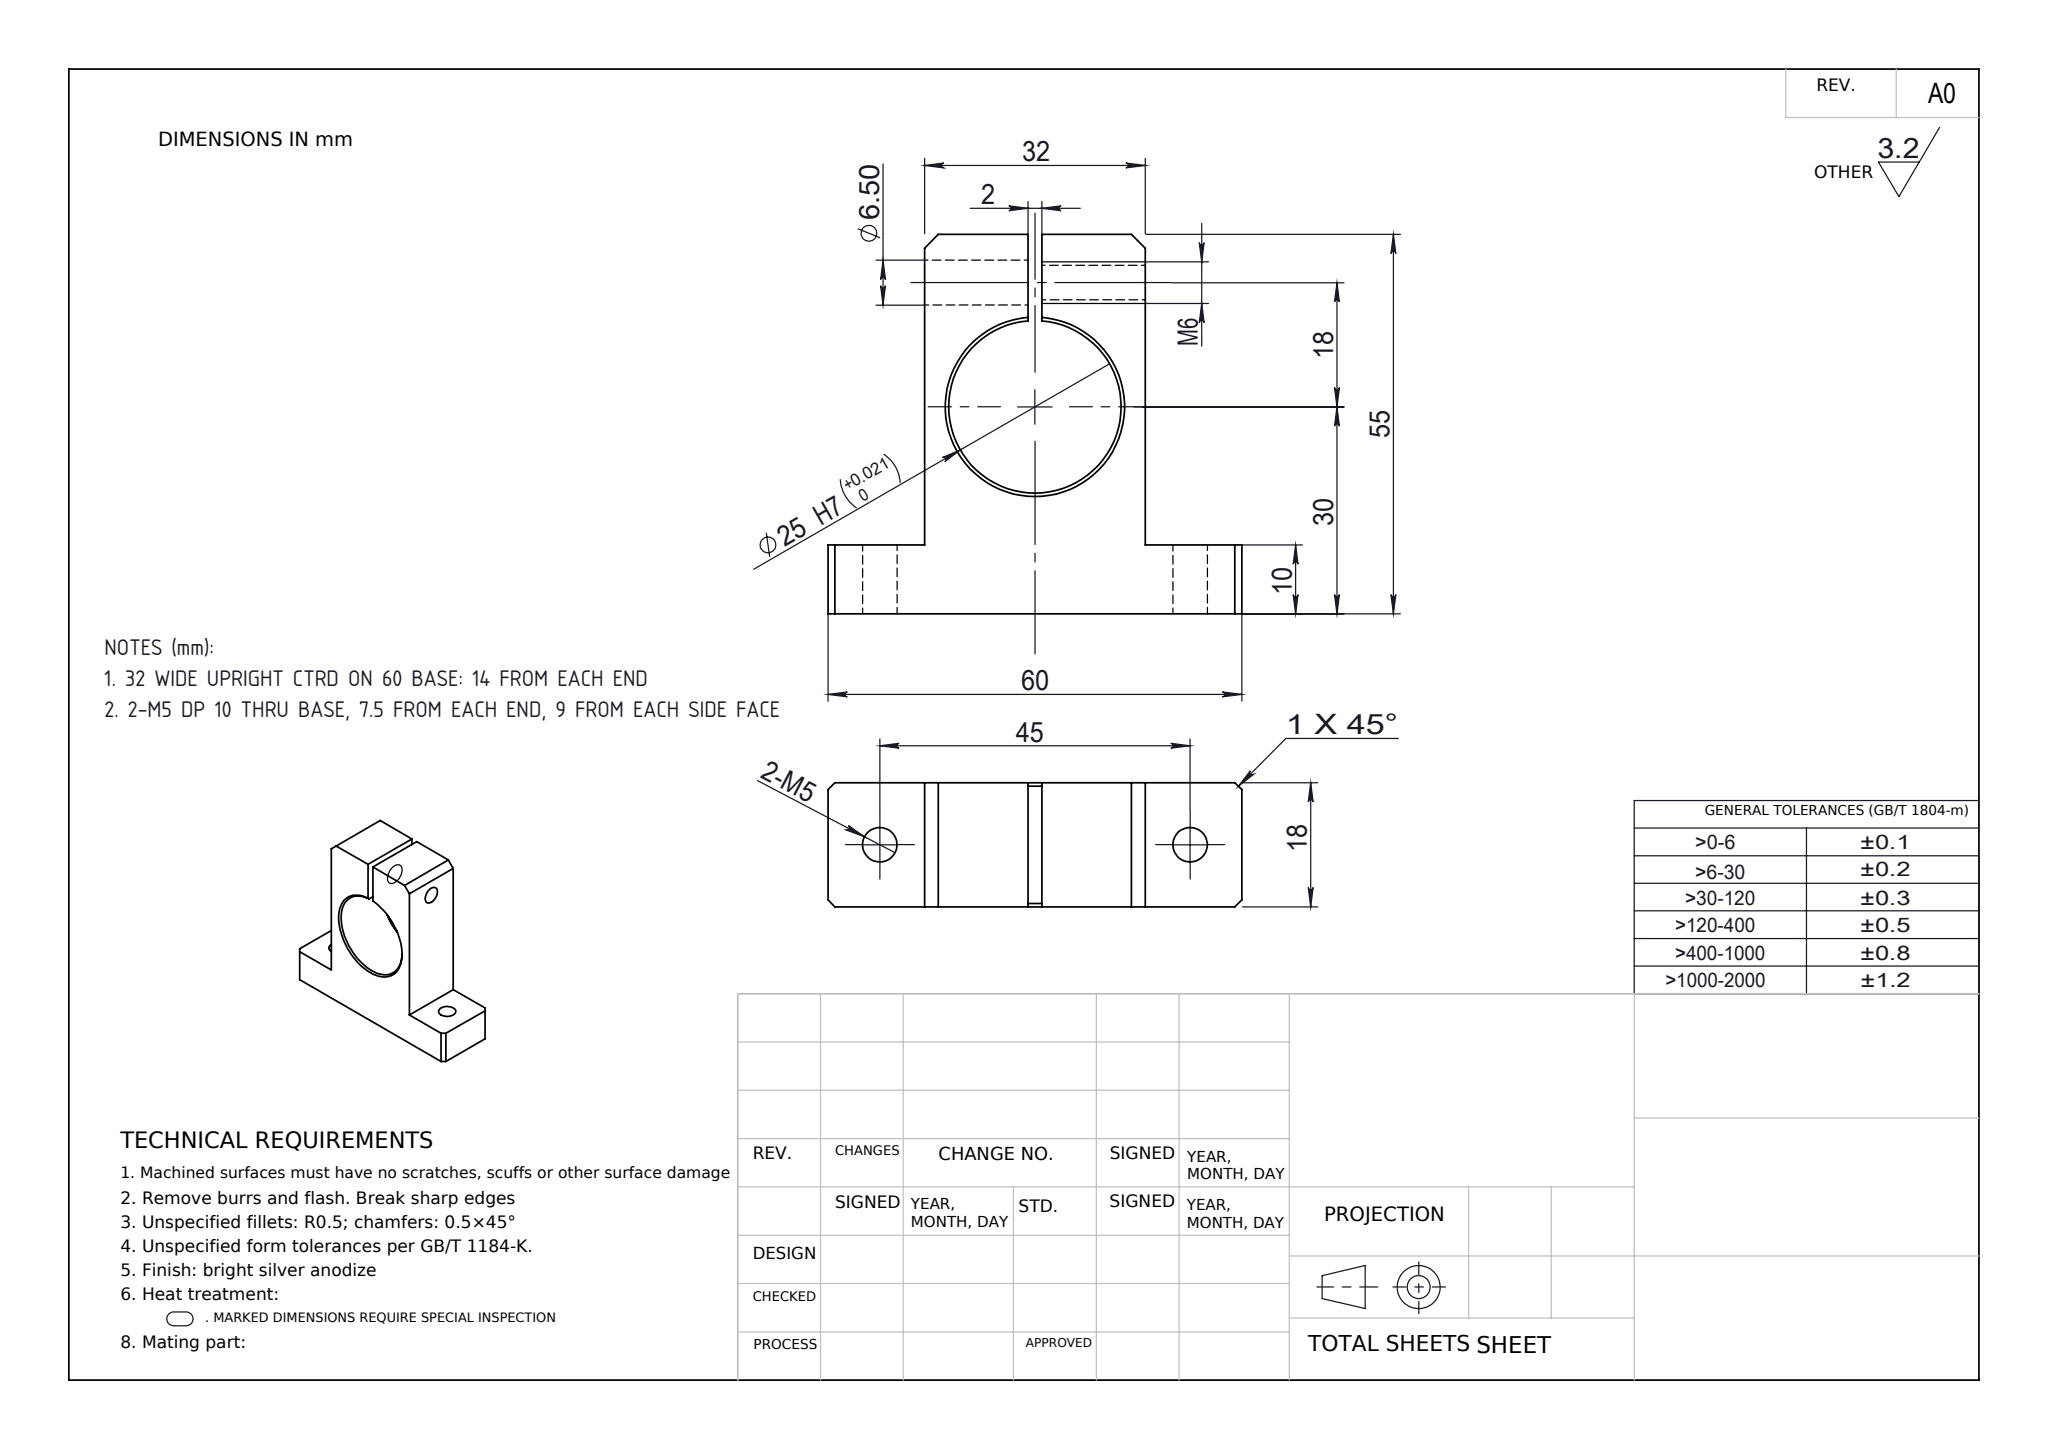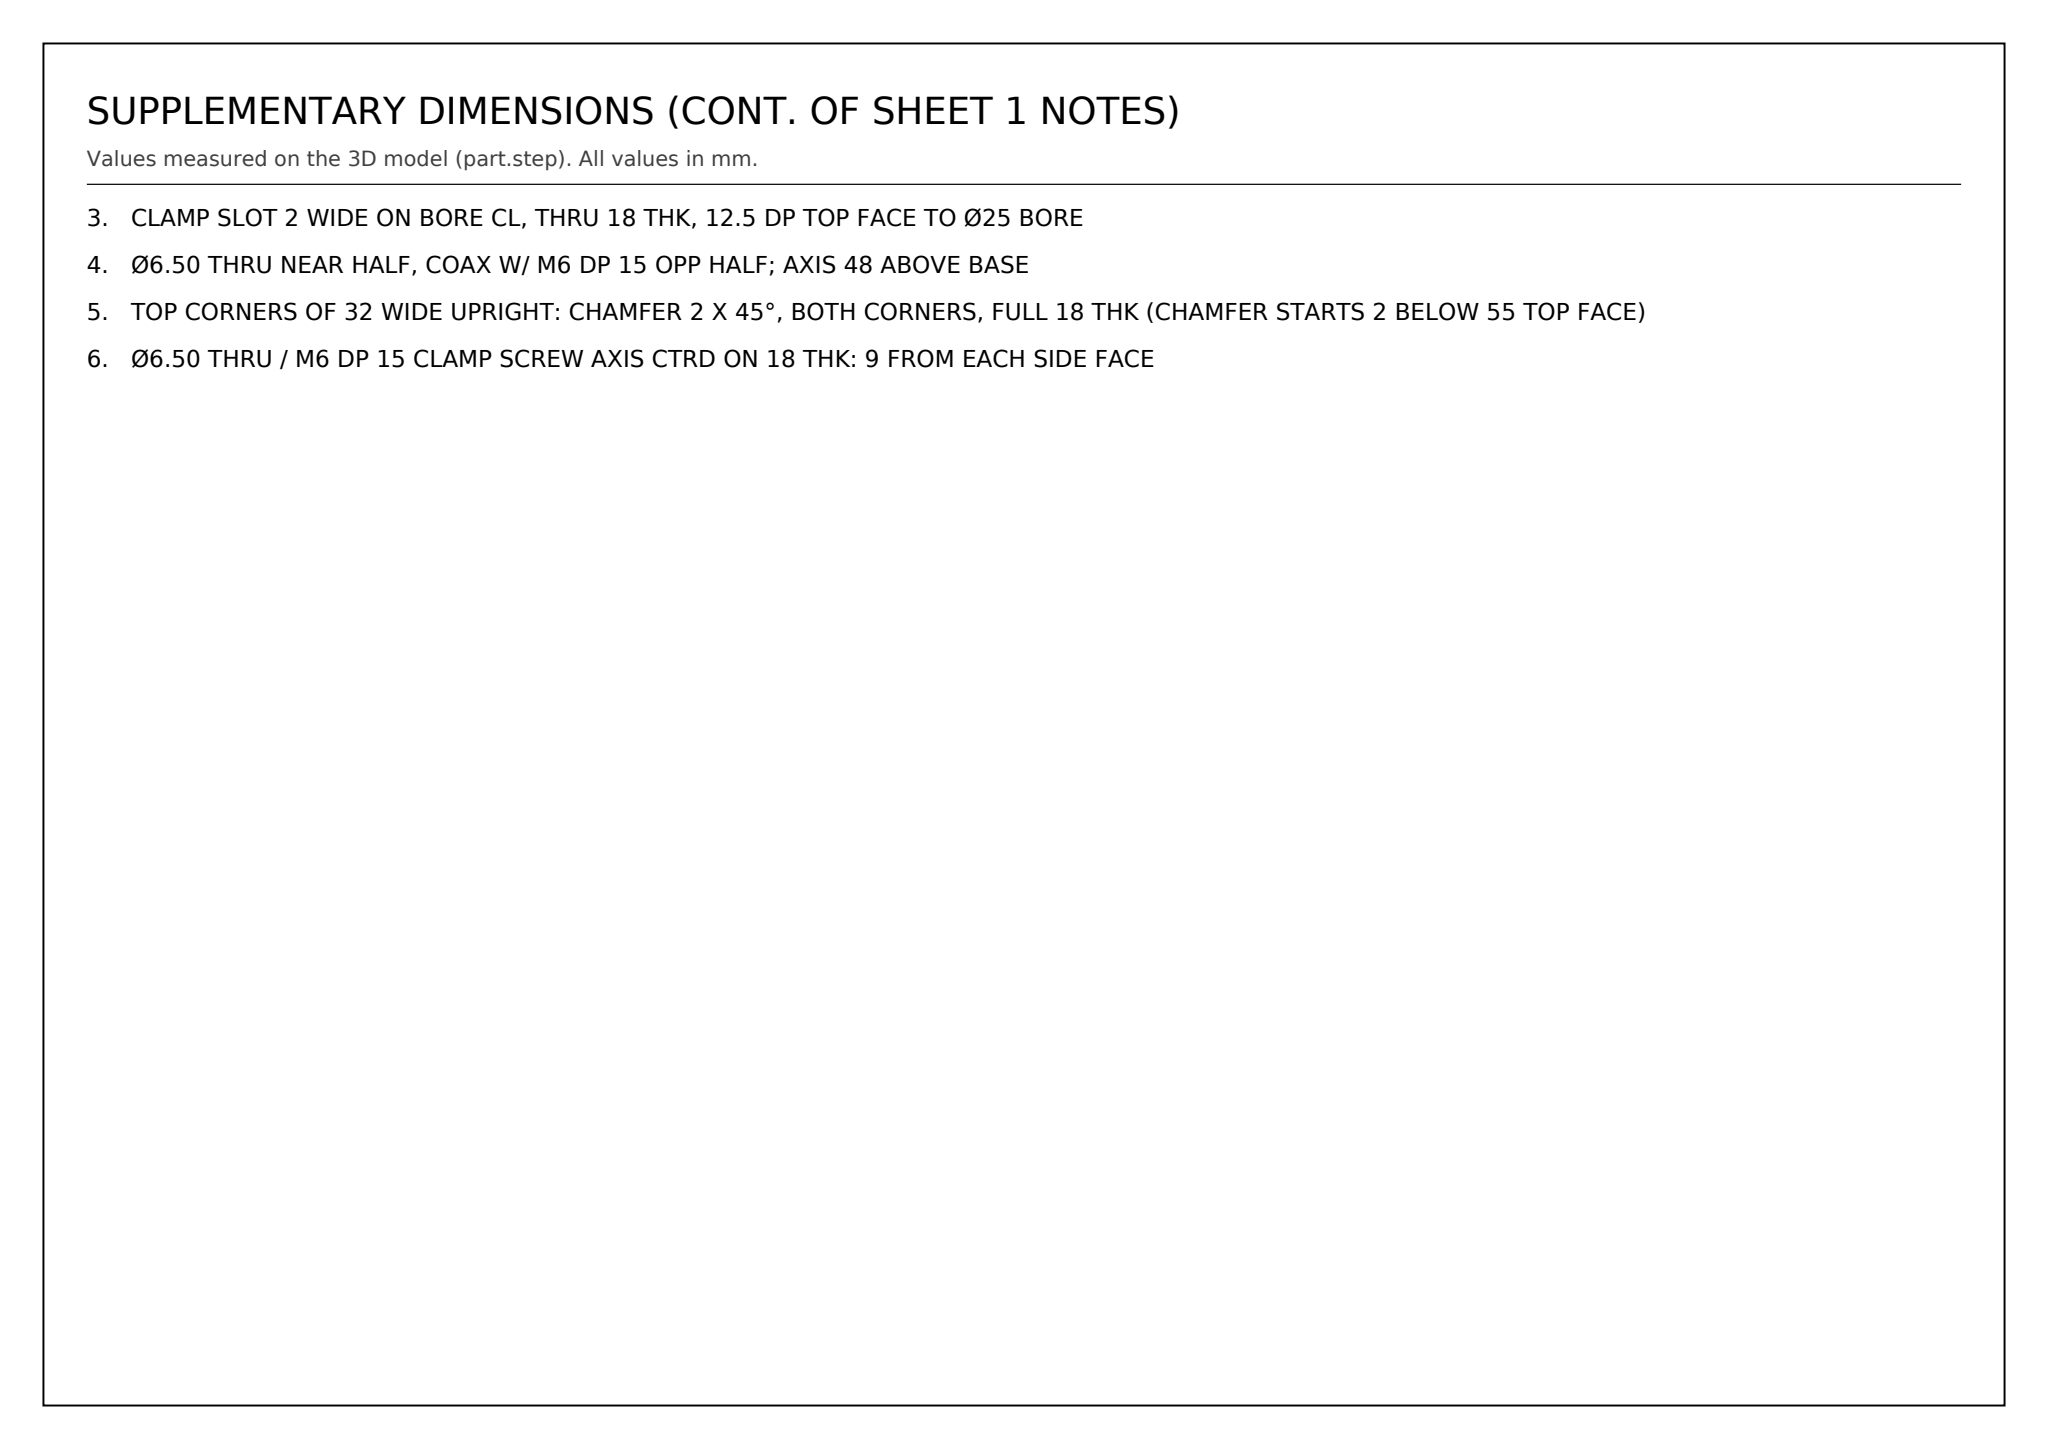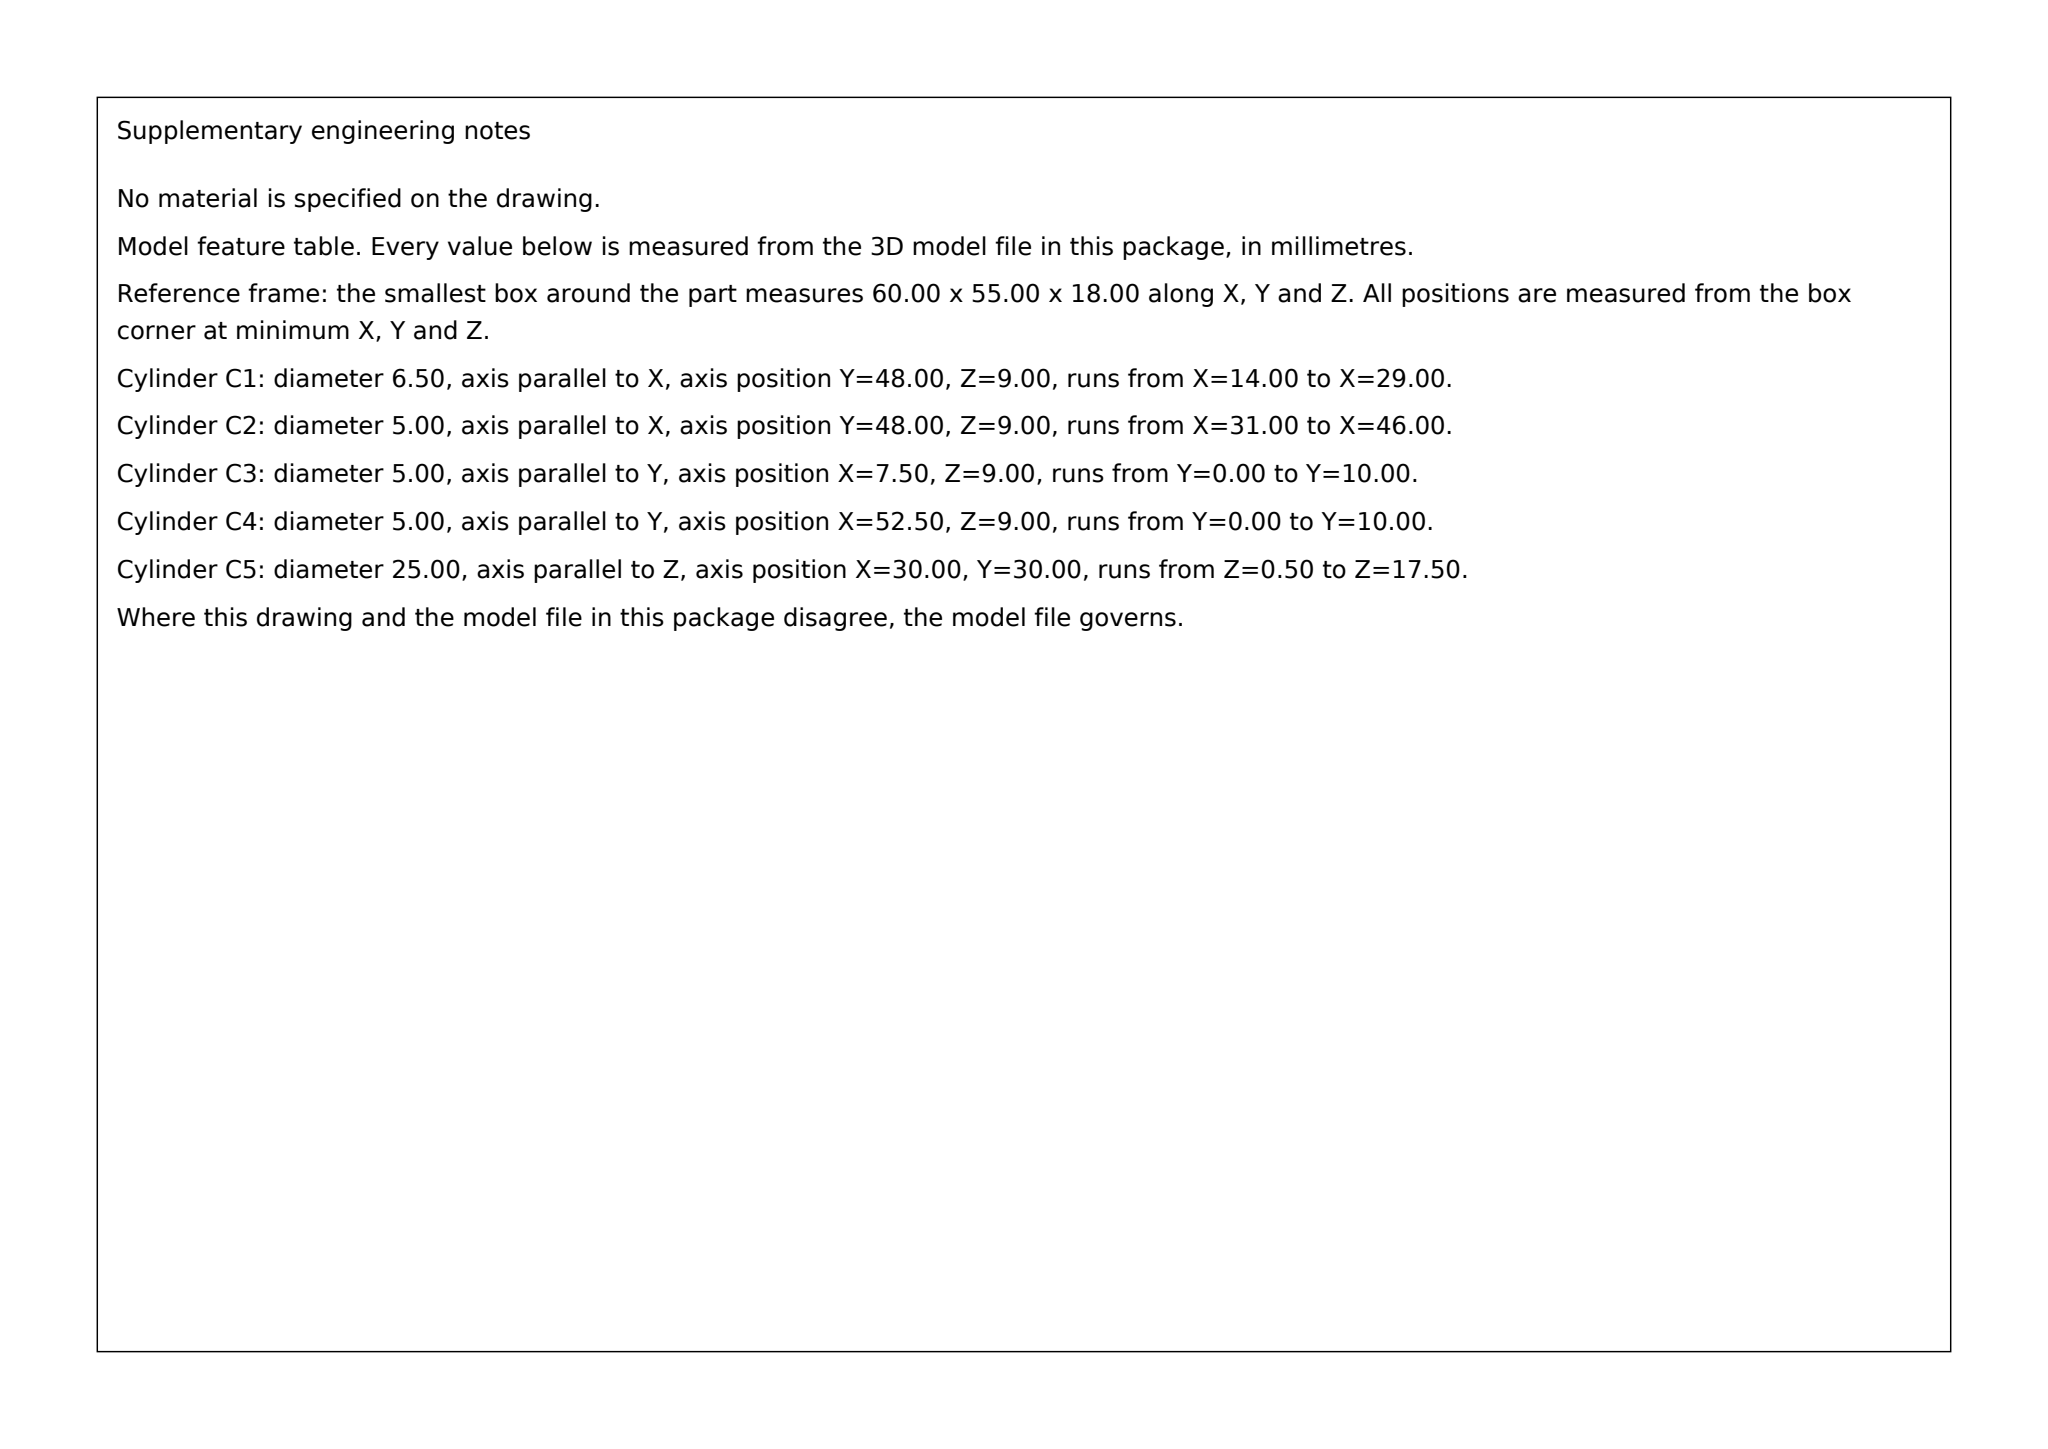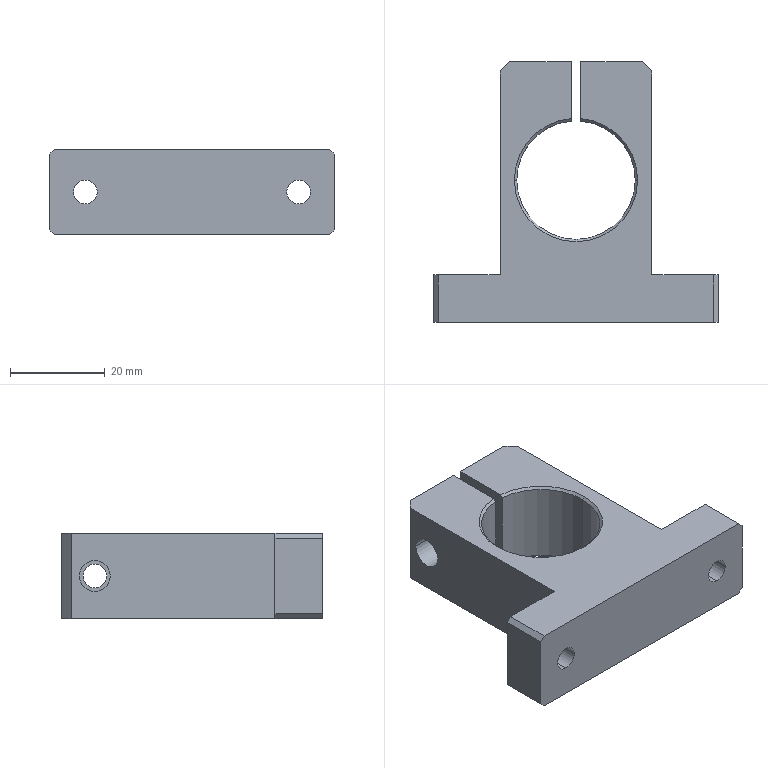Part | SolidWorks | mm | 1 solid | 36 faces | box 60 x 55 x 18 mm | volume 26137 mm3 | plane 19 | cylinder 11 | cone 6 | commonest cylinder face diameters 5 x6 25 x3 6.5 x2
Drawing notes:
32 WIDE UPRIGHT CTRD ON 60 BASE: 14 FROM EACH END | from the solid: x-planes at 14 and 46 vs bbox x 0-60
2-M5 DP 10 THRU BASE, 7.5 FROM EACH END, 9 FROM EACH SIDE FACE | from the solid: cyl Ø5 axis y at x=7.5 & x=52.5, z=9, length 10; base 60 long x 18 wide
CLAMP SLOT 2 WIDE ON BORE CL, THRU 18 THK, 12.5 DP TOP FACE TO Ø25 BORE | from the solid: x-planes 29 & 31 (2 wide, ctr x=30 bore axis); z 0-18 full thk; top y=55 to bore top y=42.5
Ø6.50 THRU NEAR HALF, COAX W/ M6 DP 15 OPP HALF; AXIS 48 ABOVE BASE | from the solid: Ø6.5 and Ø5 cyls, axis X, pos y=48 z=9, length 15 ea; halves x14-29 and x31-46; bbox ht 55
TOP CORNERS OF 32 WIDE UPRIGHT: CHAMFER 2 X 45°, BOTH CORNERS, FULL 18 THK (CHAMFER STARTS 2 BELOW 55 TOP FACE) | from the solid: inclined_planes: two 45°/45° faces, bbox_from [14,53,0] and [44,53,0], size [2,2,18]
Ø6.50 THRU / M6 DP 15 CLAMP SCREW AXIS CTRD ON 18 THK: 9 FROM EACH SIDE FACE | from the solid: cylinders: Ø6.50 x-axis at [y 48, z 9] from x14 to x29 and Ø5.0 (M6) x-axis at [y 48, z 9] from x31 to x46; bbox z = 18
build123d program:
from build123d import *

# Parameters (mm, degrees)
EXTRUDE1_DEPTH     = 9
CHAMFER1_SIZE      = 2
SKETCH4_R          = 3.25
CUT_EXTRUDE3_DEPTH = 64.773
CHAMFER1_2_SIZE    = 1
M5_TAPPED_HOLE1_D  = 5
CHAMFER2_SIZE      = 0.5
M6_TAPPED_HOLE1_D  = 5


with BuildPart() as part:
    # Sketch1 → Extrude1 (new, symmetric)
    with BuildSketch(Plane.XY):
        with BuildLine():
            Line((16, 55), (1, 55))
            Line((1, 55), (1, 42.46))
            ThreePointArc((1, 42.46), (0, 17.5), (-1, 42.46))
            Line((-1, 42.46), (-1, 55))
            Line((-1, 55), (-16, 55))
            Line((-16, 55), (-16, 10))
            Line((-16, 10), (-30, 10))
            Line((-30, 10), (-30, 0))
            Line((-30, 0), (30, 0))
            Line((30, 0), (30, 10))
            Line((30, 10), (16, 10))
            Line((16, 10), (16, 55))
        make_face()
    extrude(amount=EXTRUDE1_DEPTH, both=True)

    # Chamfer1
    chamfer1_edges = [part.edges().sort_by_distance(p)[0] for p in [
        (16, 55, 0),
        (-16, 55, 0),
    ]]
    chamfer(chamfer1_edges, length=CHAMFER1_SIZE)

    # Sketch4 → Cut-Extrude3 (cut, through all)
    with BuildSketch(Plane(origin=(-1, 0, 0), x_dir=(0, 0, -1), z_dir=(1, 0, 0))):
        with Locations(Location((0, 48, 0), (0, 0, 90))):
            Circle(SKETCH4_R)
    extrude(amount=-CUT_EXTRUDE3_DEPTH, mode=Mode.SUBTRACT)

    # Chamfer1_2
    chamfer1_2_edges = [part.edges().sort_by_distance(p)[0] for p in [
        (-30, 5, 9),
        (30, 5, -9),
        (-30, 5, -9),
        (30, 5, 9),
    ]]
    chamfer(chamfer1_2_edges, length=CHAMFER1_2_SIZE)

    # M5 Tapped Hole1 (through all)
    with Locations(Plane(origin=(0, 10, 0), x_dir=(-1, 0, 0), z_dir=(0, 1, 0))):
        with Locations((22.5, 0), (-22.5, 0)):
            Hole(M5_TAPPED_HOLE1_D / 2)

    # Chamfer2
    chamfer2_edges = [part.edges().sort_by_distance(p)[0] for p in [
        (0, 17.5, -9),
        (0, 17.5, 9),
    ]]
    chamfer(chamfer2_edges, length=CHAMFER2_SIZE)

    # M6 Tapped Hole1 (through all)
    with Locations(Plane.ZY.offset(-1)):
        with Locations((0, 48)):
            Hole(M6_TAPPED_HOLE1_D / 2)


solid = part.part